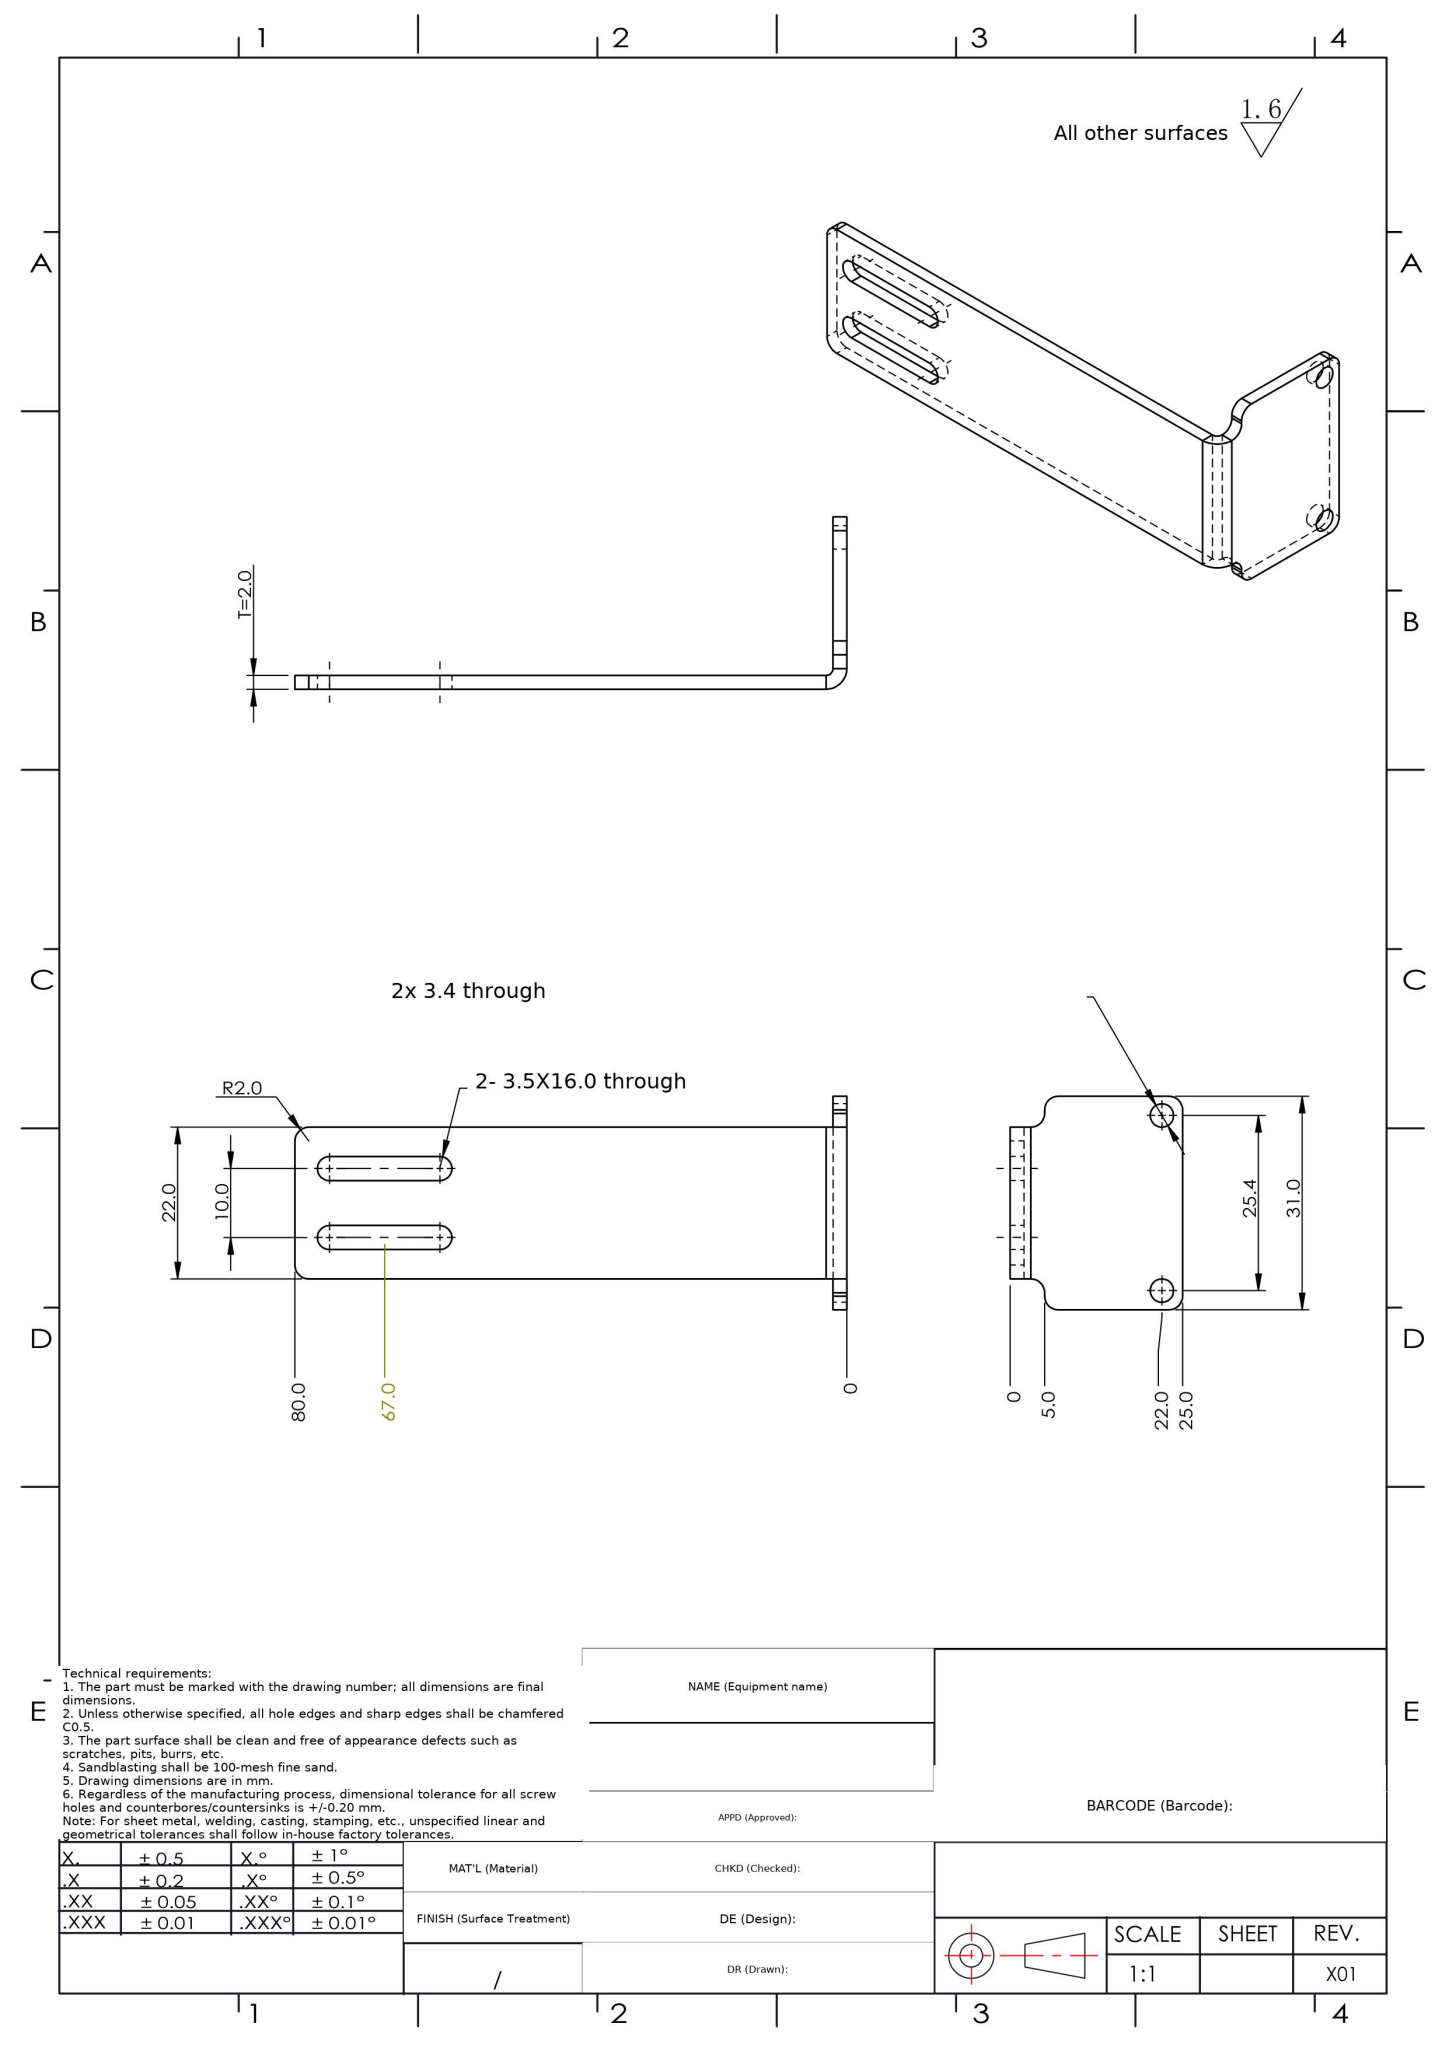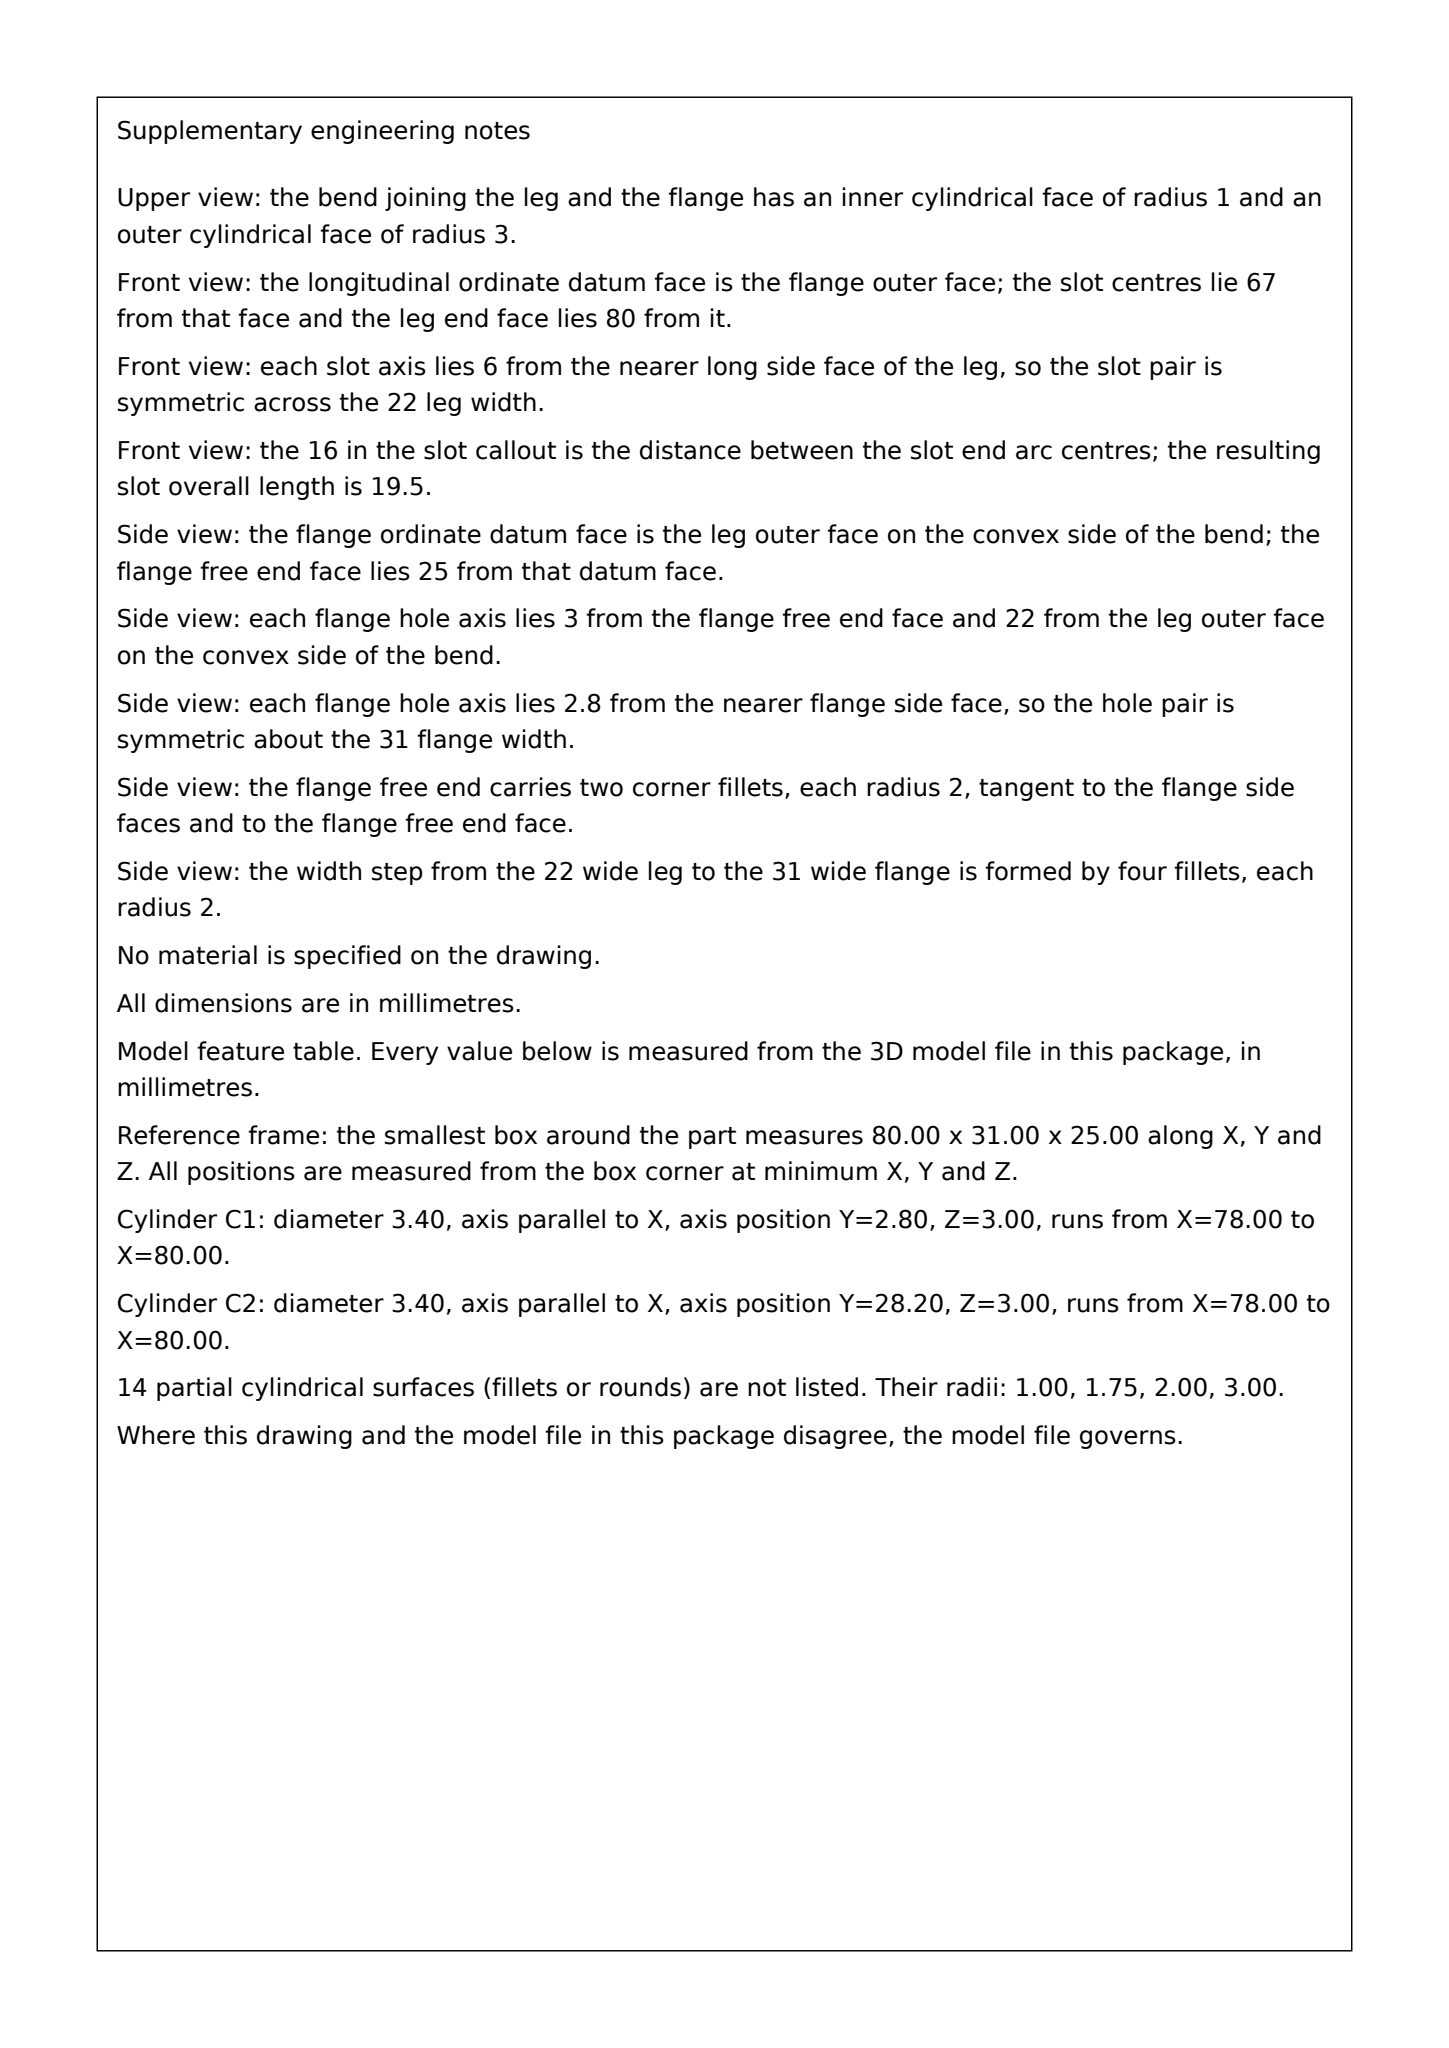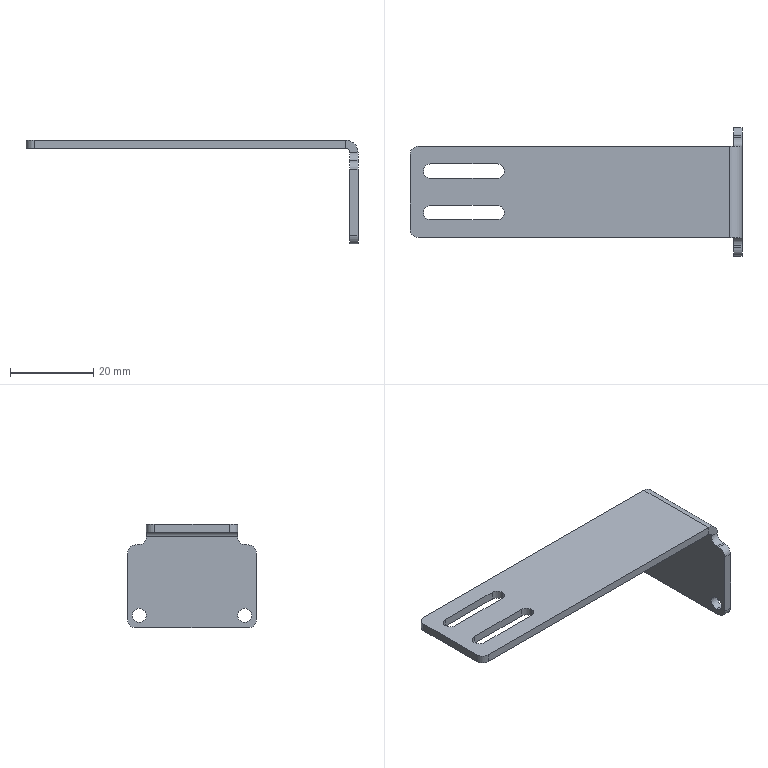Part | SolidWorks | mm | 1 solid | 38 faces | box 80 x 31 x 25 mm | volume 4549 mm3 | cylinder 20 | plane 18 | commonest cylinder face diameters 4 x8 3.5 x6 3.4 x4 6 x1 2 x1
Drawing notes:
4: 2X 3.5X16.0 SLOT, CL 6.0 FROM EACH LONG EDGE OF 22.0 FACE | from the solid: 3.5 dia z-axis slot ends at y=10.5 & 20.5; flange faces y=4.5 & 26.5 -> 6.0 each side
5: 2X Ø3.4 THRU, CL 2.8 FROM EDGE; 25.4 APART ON 31.0 FACE | from the solid: 3.4 dia x-axis holes at y=2.8 and y=28.2; face y=0 to 31.0 -> 2.8 edge dist, 25.4 spacing